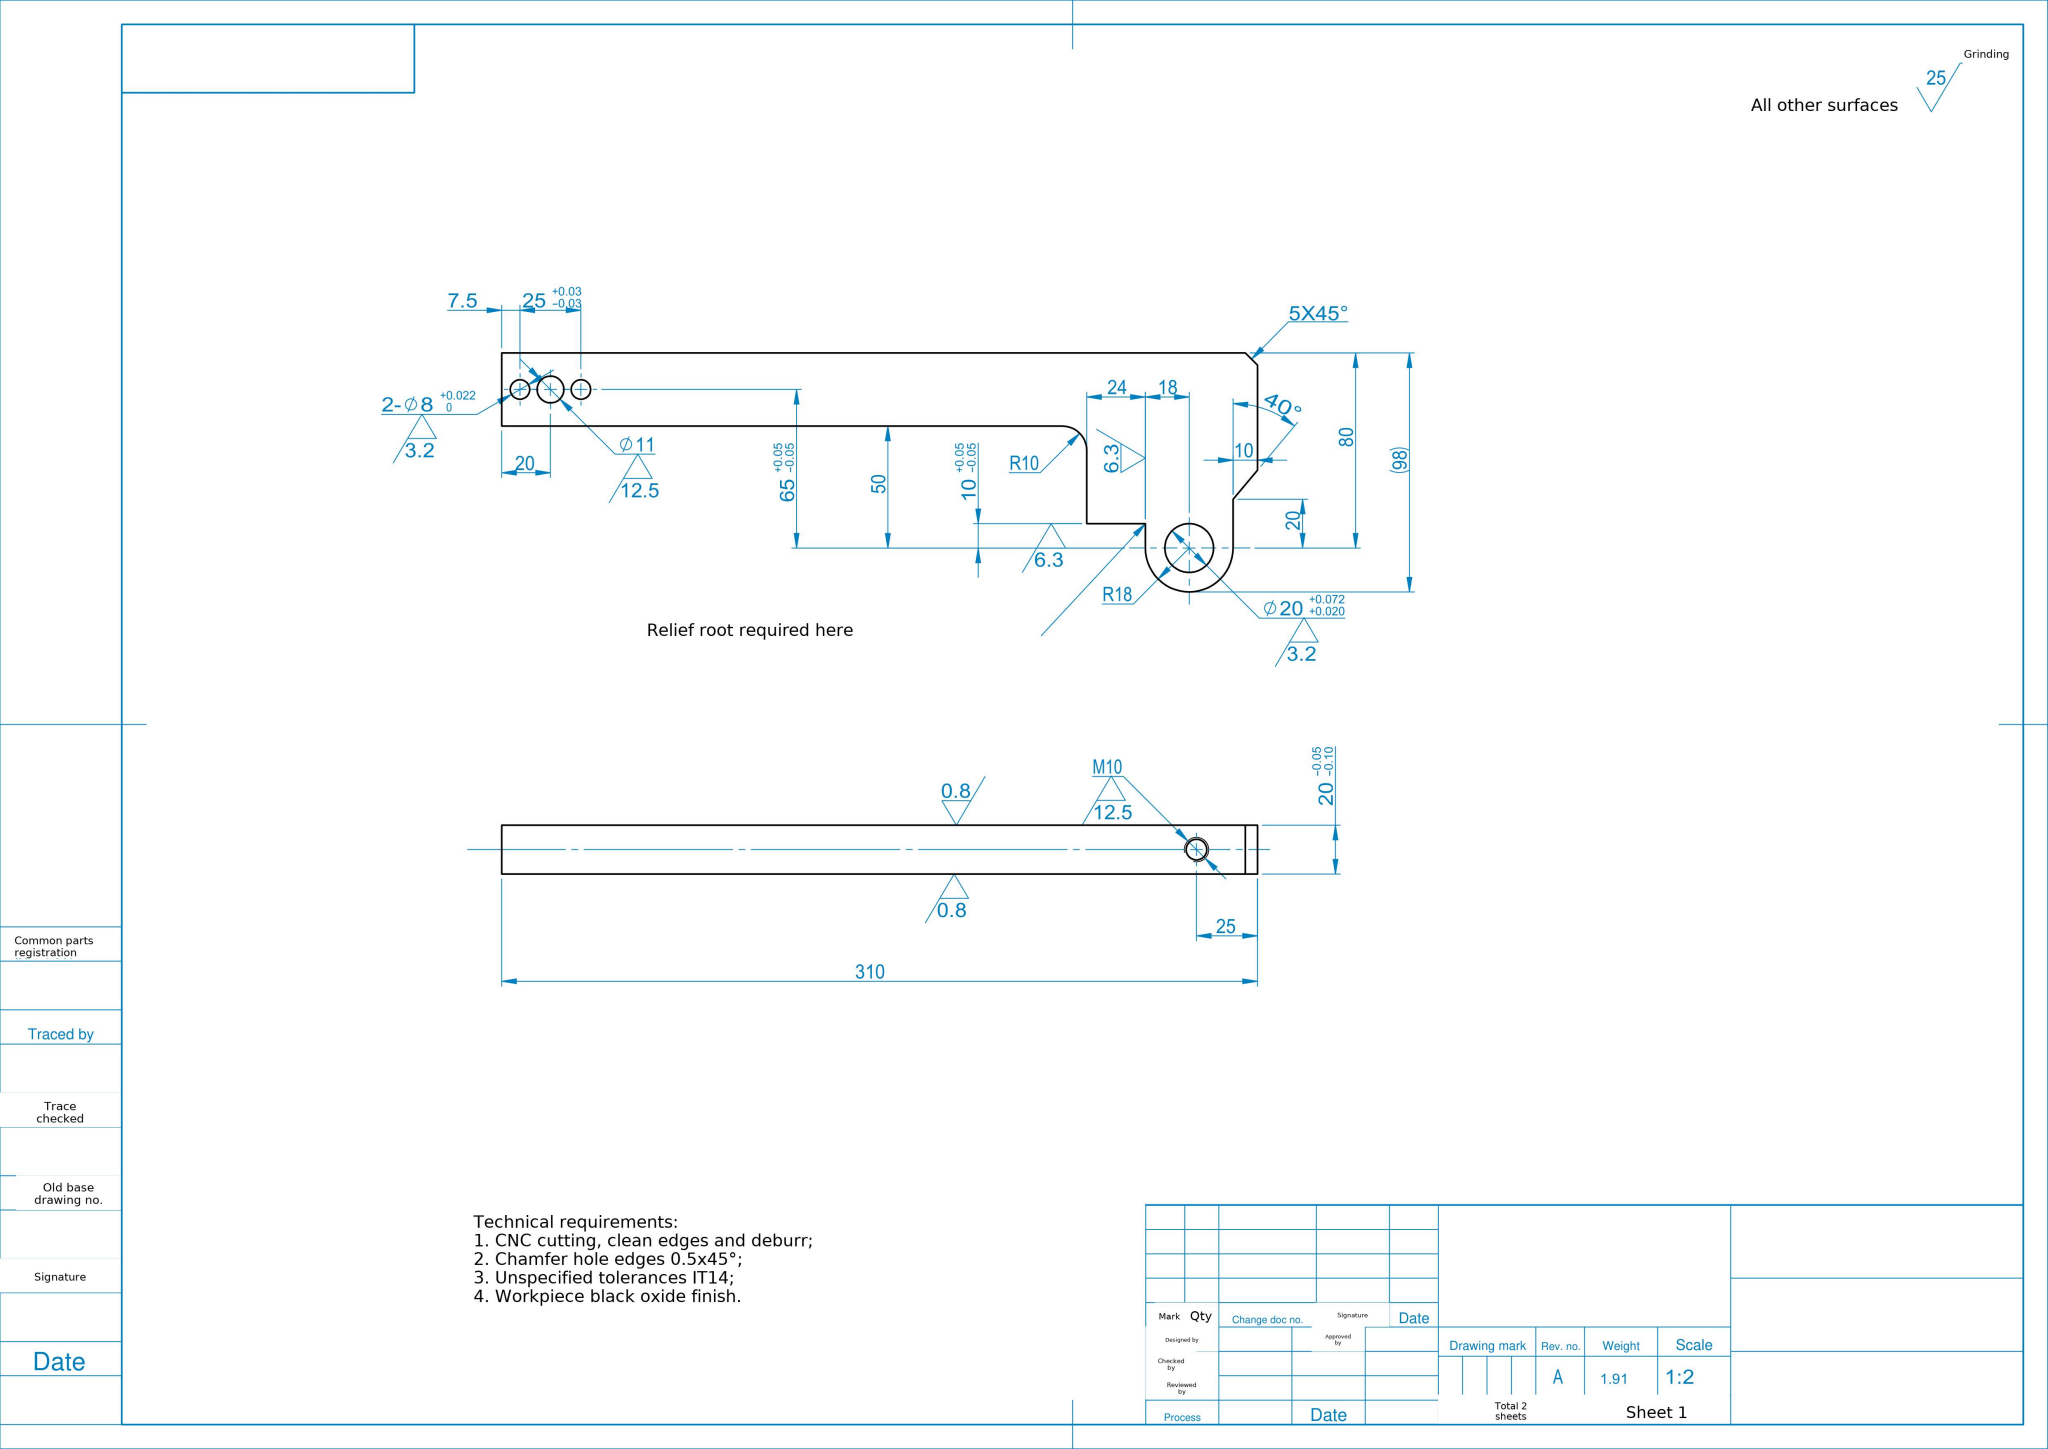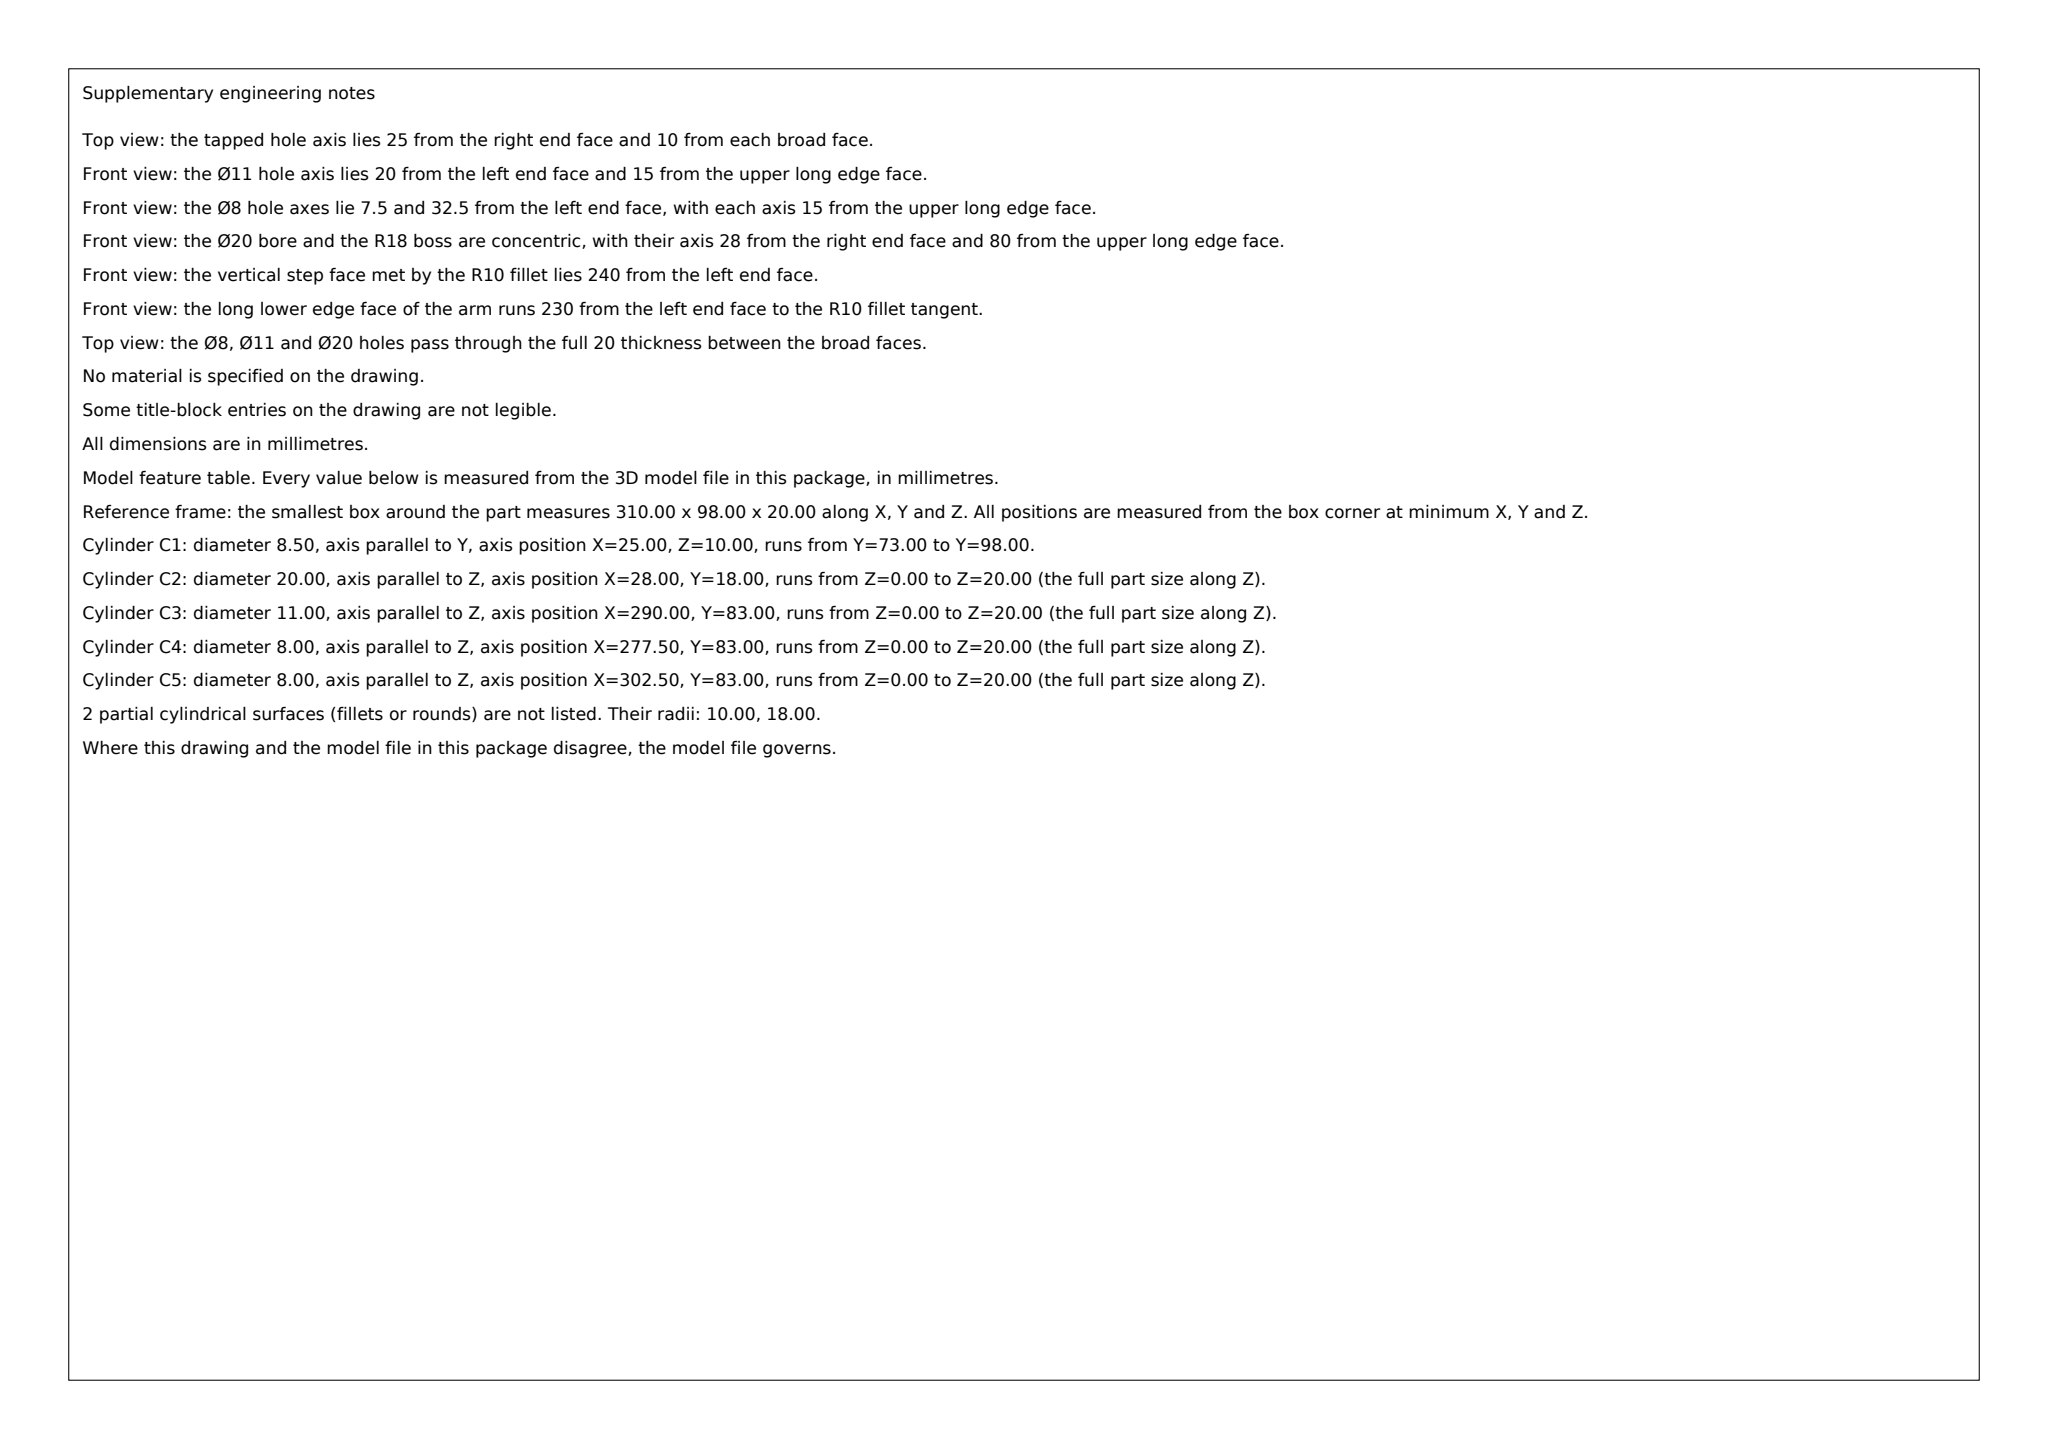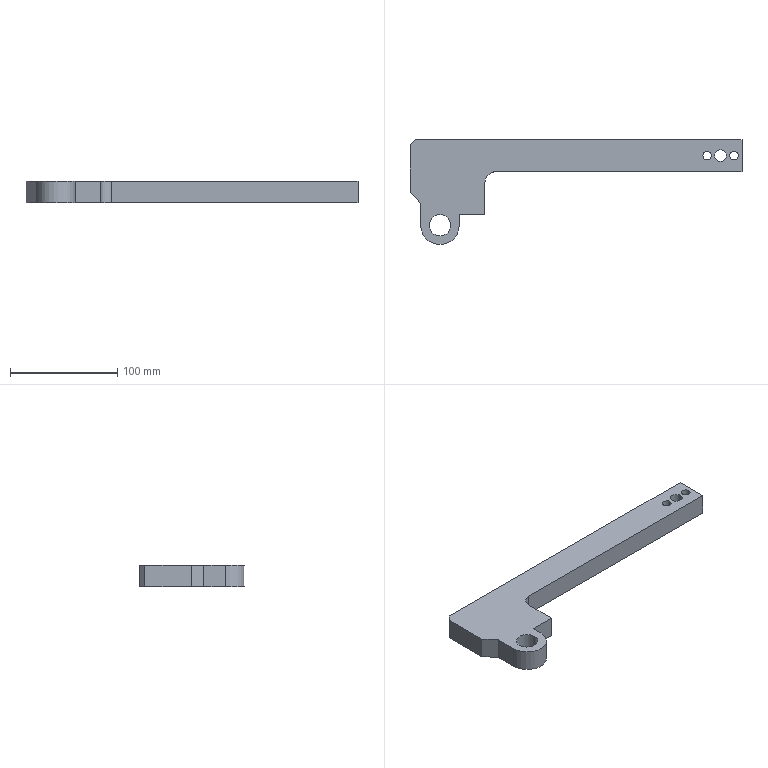Part | SolidWorks | mm | 1 solid | 26 faces | box 310 x 98 x 20 mm | volume 244705 mm3 | cylinder 12 | plane 12 | cone 2 | commonest cylinder face diameters 8 x4 20 x3 11 x2 8.5 x2 36 x1
Drawing notes:
M10 DP 25; Ø8.5 DRILL DP 25, 118° PT (FROM Ø20 BOSS END FACE) | from the solid: cylinder [8.5,"y",[25.0,null,10.0],25.0] blind from y=98 face; cone 118° ref dia 8.5
build123d program:
from build123d import *

# Parameters (mm, degrees)
BOSS_EXTRUDE1_DEPTH    = 20
SKETCH2_R              = 10
CUT_EXTRUDE1_DEPTH     = 319
M10_TAPPED_HOLE1_D     = 8.5
M10_TAPPED_HOLE1_DEPTH = 25
M10_TAPPED_HOLE1_TIP   = 2.554
CHAMFER1_SIZE          = 5
SKETCH8_R              = 5.5
CUT_EXTRUDE2_DEPTH     = 319
SKETCH9_R              = 4
CUT_EXTRUDE3_DEPTH     = 319
FILLET1_R              = 10


with BuildPart() as part:
    # Sketch1 → Boss-Extrude1 (new body)
    with BuildSketch(Plane.XY):
        with BuildLine():
            Line((-264, -40), (-264, -50))
            ThreePointArc((-264, -50), (-282, -68), (-300, -50))
            Line((-300, -50), (-300, -30))
            Line((-300, -30), (-310, -18.082))
            Line((-310, -18.082), (-310, 30))
            Line((-310, 30), (0, 30))
            Line((0, 30), (0, 0))
            Line((0, 0), (-240, 0))
            Line((-240, 0), (-240, -40))
            Line((-240, -40), (-264, -40))
        make_face()
    extrude(amount=BOSS_EXTRUDE1_DEPTH)

    # Sketch2 → Cut-Extrude1 (cut, through all)
    with BuildSketch(Plane(origin=(0, 0, 0), x_dir=(-1, 0, 0), z_dir=(0, 0, -1))):
        with Locations((282, -50)):
            Circle(SKETCH2_R)
    extrude(amount=-CUT_EXTRUDE1_DEPTH, mode=Mode.SUBTRACT)

    # M10 Tapped Hole1
    with Locations(Plane(origin=(0, 30, 0), x_dir=(1, 0, 0), z_dir=(0, 1, 0))):
        with Locations((-285, -10)):
            Hole(M10_TAPPED_HOLE1_D / 2, depth=M10_TAPPED_HOLE1_DEPTH)
            with Locations((0, 0, -(M10_TAPPED_HOLE1_DEPTH + M10_TAPPED_HOLE1_TIP / 2))):  # 118° drill point
                Cone(0, M10_TAPPED_HOLE1_D / 2, M10_TAPPED_HOLE1_TIP, mode=Mode.SUBTRACT)

    # Chamfer1
    chamfer1_edges = [part.edges().sort_by_distance(p)[0] for p in [
        (-310, 30, 10),
    ]]
    chamfer(chamfer1_edges, length=CHAMFER1_SIZE)

    # Sketch8 → Cut-Extrude2 (cut, through all)
    with BuildSketch(Plane(origin=(0, 0, 0), x_dir=(-1, 0, 0), z_dir=(0, 0, -1))):
        with Locations((20, 15)):
            Circle(SKETCH8_R)
    extrude(amount=-CUT_EXTRUDE2_DEPTH, mode=Mode.SUBTRACT)

    # Sketch9 → Cut-Extrude3 (cut, through all)
    with BuildSketch(Plane(origin=(0, 0, 0), x_dir=(-1, 0, 0), z_dir=(0, 0, -1))):
        with Locations((7.5, 15)):
            Circle(SKETCH9_R)
        with Locations((32.5, 15)):
            Circle(SKETCH9_R)
    extrude(amount=-CUT_EXTRUDE3_DEPTH, mode=Mode.SUBTRACT)

    # Fillet1
    fillet1_edges = [part.edges().sort_by_distance(p)[0] for p in [
        (-240, 0, 10),
    ]]
    fillet(fillet1_edges, radius=FILLET1_R)


solid = part.part
STEP:
#1=CARTESIAN_POINT('',(-28.5,15.,20.));
#2=VERTEX_POINT('',#1);
#3=CARTESIAN_POINT('',(-36.5,15.,20.));
#4=VERTEX_POINT('',#3);
#5=CARTESIAN_POINT('',(-32.5,15.,20.));
#6=DIRECTION('',(0.,0.,-1.));
#7=DIRECTION('',(-1.,0.,0.));
#8=AXIS2_PLACEMENT_3D('',#5,#6,#7);
#9=CIRCLE('',#8,4.);
#10=EDGE_CURVE('',#2,#4,#9,.T.);
#11=ORIENTED_EDGE('',*,*,#10,.F.);
#12=CARTESIAN_POINT('',(-28.5,15.,0.));
#13=VERTEX_POINT('',#12);
#14=CARTESIAN_POINT('',(-28.5,15.,20.));
#15=DIRECTION('',(0.,0.,-1.));
#16=VECTOR('',#15,1000.);
#17=LINE('',#14,#16);
#18=EDGE_CURVE('',#2,#13,#17,.T.);
#19=ORIENTED_EDGE('',*,*,#18,.T.);
#20=CARTESIAN_POINT('',(-36.5,15.,0.));
#21=VERTEX_POINT('',#20);
#22=CARTESIAN_POINT('',(-32.5,15.,0.));
#23=DIRECTION('',(0.,0.,-1.));
#24=DIRECTION('',(-1.,0.,0.));
#25=AXIS2_PLACEMENT_3D('',#22,#23,#24);
#26=CIRCLE('',#25,4.);
#27=EDGE_CURVE('',#13,#21,#26,.T.);
#28=ORIENTED_EDGE('',*,*,#27,.T.);
#29=CARTESIAN_POINT('',(-36.5,15.,20.));
#30=DIRECTION('',(0.,0.,-1.));
#31=VECTOR('',#30,1000.);
#32=LINE('',#29,#31);
#33=EDGE_CURVE('',#4,#21,#32,.T.);
#34=ORIENTED_EDGE('',*,*,#33,.F.);
#35=EDGE_LOOP('',(#11,#19,#28,#34));
#36=FACE_OUTER_BOUND('',#35,.T.);
#37=CARTESIAN_POINT('',(-32.5,15.,20.));
#38=DIRECTION('',(0.,0.,-1.));
#39=DIRECTION('',(-1.,0.,0.));
#40=AXIS2_PLACEMENT_3D('',#37,#38,#39);
#41=CYLINDRICAL_SURFACE('',#40,4.);
#42=ADVANCED_FACE('',(#36),#41,.F.);
#43=CARTESIAN_POINT('',(-3.5,15.,20.));
#44=VERTEX_POINT('',#43);
#45=CARTESIAN_POINT('',(-11.5,15.,20.));
#46=VERTEX_POINT('',#45);
#47=CARTESIAN_POINT('',(-7.5,15.,20.));
#48=DIRECTION('',(0.,0.,-1.));
#49=DIRECTION('',(-1.,0.,0.));
#50=AXIS2_PLACEMENT_3D('',#47,#48,#49);
#51=CIRCLE('',#50,4.);
#52=EDGE_CURVE('',#44,#46,#51,.T.);
#53=ORIENTED_EDGE('',*,*,#52,.F.);
#54=CARTESIAN_POINT('',(-3.5,15.,0.));
#55=VERTEX_POINT('',#54);
#56=CARTESIAN_POINT('',(-3.5,15.,20.));
#57=DIRECTION('',(0.,0.,-1.));
#58=VECTOR('',#57,1000.);
#59=LINE('',#56,#58);
#60=EDGE_CURVE('',#44,#55,#59,.T.);
#61=ORIENTED_EDGE('',*,*,#60,.T.);
#62=CARTESIAN_POINT('',(-11.5,15.,0.));
#63=VERTEX_POINT('',#62);
#64=CARTESIAN_POINT('',(-7.5,15.,0.));
#65=DIRECTION('',(0.,0.,-1.));
#66=DIRECTION('',(-1.,0.,0.));
#67=AXIS2_PLACEMENT_3D('',#64,#65,#66);
#68=CIRCLE('',#67,4.);
#69=EDGE_CURVE('',#55,#63,#68,.T.);
#70=ORIENTED_EDGE('',*,*,#69,.T.);
#71=CARTESIAN_POINT('',(-11.5,15.,20.));
#72=DIRECTION('',(0.,0.,-1.));
#73=VECTOR('',#72,1000.);
#74=LINE('',#71,#73);
#75=EDGE_CURVE('',#46,#63,#74,.T.);
#76=ORIENTED_EDGE('',*,*,#75,.F.);
#77=EDGE_LOOP('',(#53,#61,#70,#76));
#78=FACE_OUTER_BOUND('',#77,.T.);
#79=CARTESIAN_POINT('',(-7.5,15.,20.));
#80=DIRECTION('',(0.,0.,-1.));
#81=DIRECTION('',(-1.,0.,0.));
#82=AXIS2_PLACEMENT_3D('',#79,#80,#81);
#83=CYLINDRICAL_SURFACE('',#82,4.);
#84=ADVANCED_FACE('',(#78),#83,.F.);
#85=CARTESIAN_POINT('',(-14.5,15.,20.));
#86=VERTEX_POINT('',#85);
#87=CARTESIAN_POINT('',(-25.5,15.,20.));
#88=VERTEX_POINT('',#87);
#89=CARTESIAN_POINT('',(-20.,15.,20.));
#90=DIRECTION('',(0.,0.,-1.));
#91=DIRECTION('',(-1.,0.,0.));
#92=AXIS2_PLACEMENT_3D('',#89,#90,#91);
#93=CIRCLE('',#92,5.5);
#94=EDGE_CURVE('',#86,#88,#93,.T.);
#95=ORIENTED_EDGE('',*,*,#94,.F.);
#96=CARTESIAN_POINT('',(-14.5,15.,0.));
#97=VERTEX_POINT('',#96);
#98=CARTESIAN_POINT('',(-14.5,15.,20.));
#99=DIRECTION('',(0.,0.,-1.));
#100=VECTOR('',#99,1000.);
#101=LINE('',#98,#100);
#102=EDGE_CURVE('',#86,#97,#101,.T.);
#103=ORIENTED_EDGE('',*,*,#102,.T.);
#104=CARTESIAN_POINT('',(-25.5,15.,0.));
#105=VERTEX_POINT('',#104);
#106=CARTESIAN_POINT('',(-20.,15.,0.));
#107=DIRECTION('',(0.,0.,-1.));
#108=DIRECTION('',(-1.,0.,0.));
#109=AXIS2_PLACEMENT_3D('',#106,#107,#108);
#110=CIRCLE('',#109,5.5);
#111=EDGE_CURVE('',#97,#105,#110,.T.);
#112=ORIENTED_EDGE('',*,*,#111,.T.);
#113=CARTESIAN_POINT('',(-25.5,15.,20.));
#114=DIRECTION('',(0.,0.,-1.));
#115=VECTOR('',#114,1000.);
#116=LINE('',#113,#115);
#117=EDGE_CURVE('',#88,#105,#116,.T.);
#118=ORIENTED_EDGE('',*,*,#117,.F.);
#119=EDGE_LOOP('',(#95,#103,#112,#118));
#120=FACE_OUTER_BOUND('',#119,.T.);
#121=CARTESIAN_POINT('',(-20.,15.,20.));
#122=DIRECTION('',(0.,0.,-1.));
#123=DIRECTION('',(-1.,0.,0.));
#124=AXIS2_PLACEMENT_3D('',#121,#122,#123);
#125=CYLINDRICAL_SURFACE('',#124,5.5);
#126=ADVANCED_FACE('',(#120),#125,.F.);
#127=CARTESIAN_POINT('',(-285.,5.,5.75));
#128=VERTEX_POINT('',#127);
#129=CARTESIAN_POINT('',(-285.,5.,14.25));
#130=VERTEX_POINT('',#129);
#131=CARTESIAN_POINT('',(-285.,5.,10.));
#132=DIRECTION('',(0.,1.,0.));
#133=DIRECTION('',(0.,0.,1.));
#134=AXIS2_PLACEMENT_3D('',#131,#132,#133);
#135=CIRCLE('',#134,4.25);
#136=EDGE_CURVE('',#128,#130,#135,.T.);
#137=ORIENTED_EDGE('',*,*,#136,.F.);
#138=CARTESIAN_POINT('',(-285.,30.,5.75));
#139=VERTEX_POINT('',#138);
#140=CARTESIAN_POINT('',(-285.,30.,5.75));
#141=DIRECTION('',(0.,1.,0.));
#142=VECTOR('',#141,1000.);
#143=LINE('',#140,#142);
#144=EDGE_CURVE('',#128,#139,#143,.T.);
#145=ORIENTED_EDGE('',*,*,#144,.T.);
#146=CARTESIAN_POINT('',(-285.,30.,14.25));
#147=VERTEX_POINT('',#146);
#148=CARTESIAN_POINT('',(-285.,30.,10.));
#149=DIRECTION('',(0.,1.,0.));
#150=DIRECTION('',(0.,0.,1.));
#151=AXIS2_PLACEMENT_3D('',#148,#149,#150);
#152=CIRCLE('',#151,4.25);
#153=EDGE_CURVE('',#139,#147,#152,.T.);
#154=ORIENTED_EDGE('',*,*,#153,.T.);
#155=CARTESIAN_POINT('',(-285.,30.,14.25));
#156=DIRECTION('',(0.,1.,0.));
#157=VECTOR('',#156,1000.);
#158=LINE('',#155,#157);
#159=EDGE_CURVE('',#130,#147,#158,.T.);
#160=ORIENTED_EDGE('',*,*,#159,.F.);
#161=EDGE_LOOP('',(#137,#145,#154,#160));
#162=FACE_OUTER_BOUND('',#161,.T.);
#163=CARTESIAN_POINT('',(-285.,30.,10.));
#164=DIRECTION('',(0.,1.,0.));
#165=DIRECTION('',(0.,0.,1.));
#166=AXIS2_PLACEMENT_3D('',#163,#164,#165);
#167=CYLINDRICAL_SURFACE('',#166,4.25);
#168=ADVANCED_FACE('',(#162),#167,.F.);
#169=CARTESIAN_POINT('',(-285.,2.446,10.));
#170=VERTEX_POINT('',#169);
#171=CARTESIAN_POINT('',(-285.,5.,14.25));
#172=DIRECTION('',(0.,0.515,0.8572));
#173=VECTOR('',#172,1000.);
#174=LINE('',#171,#173);
#175=EDGE_CURVE('',#170,#130,#174,.T.);
#176=ORIENTED_EDGE('',*,*,#175,.F.);
#177=CARTESIAN_POINT('',(-285.,5.,5.75));
#178=DIRECTION('',(0.,0.515,-0.8572));
#179=VECTOR('',#178,1000.);
#180=LINE('',#177,#179);
#181=EDGE_CURVE('',#170,#128,#180,.T.);
#182=ORIENTED_EDGE('',*,*,#181,.T.);
#183=ORIENTED_EDGE('',*,*,#136,.T.);
#184=EDGE_LOOP('',(#176,#182,#183));
#185=FACE_OUTER_BOUND('',#184,.T.);
#186=CARTESIAN_POINT('',(-285.,5.,10.));
#187=DIRECTION('',(0.,1.,0.));
#188=DIRECTION('',(0.,0.,1.));
#189=AXIS2_PLACEMENT_3D('',#186,#187,#188);
#190=CONICAL_SURFACE('',#189,4.25,1.03);
#191=ADVANCED_FACE('',(#185),#190,.F.);
#192=CARTESIAN_POINT('',(-272.,-50.,20.));
#193=VERTEX_POINT('',#192);
#194=CARTESIAN_POINT('',(-292.,-50.,20.));
#195=VERTEX_POINT('',#194);
#196=CARTESIAN_POINT('',(-282.,-50.,20.));
#197=DIRECTION('',(0.,0.,-1.));
#198=DIRECTION('',(-1.,0.,0.));
#199=AXIS2_PLACEMENT_3D('',#196,#197,#198);
#200=CIRCLE('',#199,10.);
#201=EDGE_CURVE('',#193,#195,#200,.T.);
#202=ORIENTED_EDGE('',*,*,#201,.F.);
#203=CARTESIAN_POINT('',(-272.,-50.,0.));
#204=VERTEX_POINT('',#203);
#205=CARTESIAN_POINT('',(-272.,-50.,20.));
#206=DIRECTION('',(0.,0.,-1.));
#207=VECTOR('',#206,1000.);
#208=LINE('',#205,#207);
#209=EDGE_CURVE('',#193,#204,#208,.T.);
#210=ORIENTED_EDGE('',*,*,#209,.T.);
#211=CARTESIAN_POINT('',(-292.,-50.,0.));
#212=VERTEX_POINT('',#211);
#213=CARTESIAN_POINT('',(-282.,-50.,0.));
#214=DIRECTION('',(0.,0.,-1.));
#215=DIRECTION('',(-1.,0.,0.));
#216=AXIS2_PLACEMENT_3D('',#213,#214,#215);
#217=CIRCLE('',#216,10.);
#218=EDGE_CURVE('',#204,#212,#217,.T.);
#219=ORIENTED_EDGE('',*,*,#218,.T.);
#220=CARTESIAN_POINT('',(-292.,-50.,20.));
#221=DIRECTION('',(0.,0.,-1.));
#222=VECTOR('',#221,1000.);
#223=LINE('',#220,#222);
#224=EDGE_CURVE('',#195,#212,#223,.T.);
#225=ORIENTED_EDGE('',*,*,#224,.F.);
#226=EDGE_LOOP('',(#202,#210,#219,#225));
#227=FACE_OUTER_BOUND('',#226,.T.);
#228=CARTESIAN_POINT('',(-282.,-50.,20.));
#229=DIRECTION('',(0.,0.,-1.));
#230=DIRECTION('',(-1.,0.,0.));
#231=AXIS2_PLACEMENT_3D('',#228,#229,#230);
#232=CYLINDRICAL_SURFACE('',#231,10.);
#233=ADVANCED_FACE('',(#227),#232,.F.);
#234=CARTESIAN_POINT('',(0.,0.,0.));
#235=VERTEX_POINT('',#234);
#236=CARTESIAN_POINT('',(0.,30.,0.));
#237=VERTEX_POINT('',#236);
#238=CARTESIAN_POINT('',(0.,0.,0.));
#239=DIRECTION('',(0.,1.,0.));
#240=VECTOR('',#239,1000.);
#241=LINE('',#238,#240);
#242=EDGE_CURVE('',#235,#237,#241,.T.);
#243=ORIENTED_EDGE('',*,*,#242,.T.);
#244=CARTESIAN_POINT('',(0.,30.,20.));
#245=VERTEX_POINT('',#244);
#246=CARTESIAN_POINT('',(0.,30.,20.));
#247=DIRECTION('',(0.,0.,-1.));
#248=VECTOR('',#247,1000.);
#249=LINE('',#246,#248);
#250=EDGE_CURVE('',#245,#237,#249,.T.);
#251=ORIENTED_EDGE('',*,*,#250,.F.);
#252=CARTESIAN_POINT('',(0.,0.,20.));
#253=VERTEX_POINT('',#252);
#254=CARTESIAN_POINT('',(0.,0.,20.));
#255=DIRECTION('',(0.,1.,0.));
#256=VECTOR('',#255,1000.);
#257=LINE('',#254,#256);
#258=EDGE_CURVE('',#253,#245,#257,.T.);
#259=ORIENTED_EDGE('',*,*,#258,.F.);
#260=CARTESIAN_POINT('',(0.,0.,20.));
#261=DIRECTION('',(0.,0.,-1.));
#262=VECTOR('',#261,1000.);
#263=LINE('',#260,#262);
#264=EDGE_CURVE('',#253,#235,#263,.T.);
#265=ORIENTED_EDGE('',*,*,#264,.T.);
#266=EDGE_LOOP('',(#243,#251,#259,#265));
#267=FACE_OUTER_BOUND('',#266,.T.);
#268=CARTESIAN_POINT('',(0.,0.,20.));
#269=DIRECTION('',(-1.,0.,0.));
#270=DIRECTION('',(0.,0.,1.));
#271=AXIS2_PLACEMENT_3D('',#268,#269,#270);
#272=PLANE('',#271);
#273=ADVANCED_FACE('',(#267),#272,.F.);
#274=CARTESIAN_POINT('',(-285.,30.,10.));
#275=DIRECTION('',(0.,1.,0.));
#276=DIRECTION('',(0.,0.,1.));
#277=AXIS2_PLACEMENT_3D('',#274,#275,#276);
#278=CIRCLE('',#277,4.25);
#279=EDGE_CURVE('',#147,#139,#278,.T.);
#280=ORIENTED_EDGE('',*,*,#279,.F.);
#281=ORIENTED_EDGE('',*,*,#153,.F.);
#282=EDGE_LOOP('',(#280,#281));
#283=FACE_BOUND('',#282,.T.);
#284=CARTESIAN_POINT('',(-305.,30.,0.));
#285=VERTEX_POINT('',#284);
#286=CARTESIAN_POINT('',(0.,30.,0.));
#287=DIRECTION('',(-1.,-0.,0.));
#288=VECTOR('',#287,1000.);
#289=LINE('',#286,#288);
#290=EDGE_CURVE('',#237,#285,#289,.T.);
#291=ORIENTED_EDGE('',*,*,#290,.T.);
#292=CARTESIAN_POINT('',(-305.,30.,20.));
#293=VERTEX_POINT('',#292);
#294=CARTESIAN_POINT('',(-305.,30.,20.));
#295=DIRECTION('',(0.,0.,1.));
#296=VECTOR('',#295,1000.);
#297=LINE('',#294,#296);
#298=EDGE_CURVE('',#285,#293,#297,.T.);
#299=ORIENTED_EDGE('',*,*,#298,.T.);
#300=CARTESIAN_POINT('',(0.,30.,20.));
#301=DIRECTION('',(-1.,-0.,0.));
#302=VECTOR('',#301,1000.);
#303=LINE('',#300,#302);
#304=EDGE_CURVE('',#245,#293,#303,.T.);
#305=ORIENTED_EDGE('',*,*,#304,.F.);
#306=ORIENTED_EDGE('',*,*,#250,.T.);
#307=EDGE_LOOP('',(#291,#299,#305,#306));
#308=FACE_OUTER_BOUND('',#307,.T.);
#309=CARTESIAN_POINT('',(0.,30.,20.));
#310=DIRECTION('',(0.,-1.,0.));
#311=DIRECTION('',(1.,0.,0.));
#312=AXIS2_PLACEMENT_3D('',#309,#310,#311);
#313=PLANE('',#312);
#314=ADVANCED_FACE('',(#283,#308),#313,.F.);
#315=CARTESIAN_POINT('',(-310.,25.,20.));
#316=VERTEX_POINT('',#315);
#317=CARTESIAN_POINT('',(-310.,-18.082,20.));
#318=VERTEX_POINT('',#317);
#319=CARTESIAN_POINT('',(-310.,30.,20.));
#320=DIRECTION('',(0.,-1.,0.));
#321=VECTOR('',#320,1000.);
#322=LINE('',#319,#321);
#323=EDGE_CURVE('',#316,#318,#322,.T.);
#324=ORIENTED_EDGE('',*,*,#323,.F.);
#325=CARTESIAN_POINT('',(-310.,25.,0.));
#326=VERTEX_POINT('',#325);
#327=CARTESIAN_POINT('',(-310.,25.,20.));
#328=DIRECTION('',(0.,0.,-1.));
#329=VECTOR('',#328,1000.);
#330=LINE('',#327,#329);
#331=EDGE_CURVE('',#316,#326,#330,.T.);
#332=ORIENTED_EDGE('',*,*,#331,.T.);
#333=CARTESIAN_POINT('',(-310.,-18.082,0.));
#334=VERTEX_POINT('',#333);
#335=CARTESIAN_POINT('',(-310.,30.,0.));
#336=DIRECTION('',(0.,-1.,0.));
#337=VECTOR('',#336,1000.);
#338=LINE('',#335,#337);
#339=EDGE_CURVE('',#326,#334,#338,.T.);
#340=ORIENTED_EDGE('',*,*,#339,.T.);
#341=CARTESIAN_POINT('',(-310.,-18.082,20.));
#342=DIRECTION('',(0.,0.,-1.));
#343=VECTOR('',#342,1000.);
#344=LINE('',#341,#343);
#345=EDGE_CURVE('',#318,#334,#344,.T.);
#346=ORIENTED_EDGE('',*,*,#345,.F.);
#347=EDGE_LOOP('',(#324,#332,#340,#346));
#348=FACE_OUTER_BOUND('',#347,.T.);
#349=CARTESIAN_POINT('',(-310.,30.,20.));
#350=DIRECTION('',(1.,0.,0.));
#351=DIRECTION('',(0.,0.,-1.));
#352=AXIS2_PLACEMENT_3D('',#349,#350,#351);
#353=PLANE('',#352);
#354=ADVANCED_FACE('',(#348),#353,.F.);
#355=CARTESIAN_POINT('',(-300.,-30.,0.));
#356=VERTEX_POINT('',#355);
#357=CARTESIAN_POINT('',(-300.,-30.,0.));
#358=DIRECTION('',(0.6428,-0.766,0.));
#359=VECTOR('',#358,1000.);
#360=LINE('',#357,#359);
#361=EDGE_CURVE('',#334,#356,#360,.T.);
#362=ORIENTED_EDGE('',*,*,#361,.T.);
#363=CARTESIAN_POINT('',(-300.,-30.,20.));
#364=VERTEX_POINT('',#363);
#365=CARTESIAN_POINT('',(-300.,-30.,20.));
#366=DIRECTION('',(0.,0.,-1.));
#367=VECTOR('',#366,1000.);
#368=LINE('',#365,#367);
#369=EDGE_CURVE('',#364,#356,#368,.T.);
#370=ORIENTED_EDGE('',*,*,#369,.F.);
#371=CARTESIAN_POINT('',(-300.,-30.,20.));
#372=DIRECTION('',(0.6428,-0.766,0.));
#373=VECTOR('',#372,1000.);
#374=LINE('',#371,#373);
#375=EDGE_CURVE('',#318,#364,#374,.T.);
#376=ORIENTED_EDGE('',*,*,#375,.F.);
#377=ORIENTED_EDGE('',*,*,#345,.T.);
#378=EDGE_LOOP('',(#362,#370,#376,#377));
#379=FACE_OUTER_BOUND('',#378,.T.);
#380=CARTESIAN_POINT('',(-300.,-30.,20.));
#381=DIRECTION('',(0.766,0.6428,0.));
#382=DIRECTION('',(-0.6428,0.766,0.));
#383=AXIS2_PLACEMENT_3D('',#380,#381,#382);
#384=PLANE('',#383);
#385=ADVANCED_FACE('',(#379),#384,.F.);
#386=CARTESIAN_POINT('',(-300.,-50.,0.));
#387=VERTEX_POINT('',#386);
#388=CARTESIAN_POINT('',(-300.,-50.,0.));
#389=DIRECTION('',(0.,-1.,0.));
#390=VECTOR('',#389,1000.);
#391=LINE('',#388,#390);
#392=EDGE_CURVE('',#356,#387,#391,.T.);
#393=ORIENTED_EDGE('',*,*,#392,.T.);
#394=CARTESIAN_POINT('',(-300.,-50.,20.));
#395=VERTEX_POINT('',#394);
#396=CARTESIAN_POINT('',(-300.,-50.,20.));
#397=DIRECTION('',(0.,0.,-1.));
#398=VECTOR('',#397,1000.);
#399=LINE('',#396,#398);
#400=EDGE_CURVE('',#395,#387,#399,.T.);
#401=ORIENTED_EDGE('',*,*,#400,.F.);
#402=CARTESIAN_POINT('',(-300.,-50.,20.));
#403=DIRECTION('',(0.,-1.,0.));
#404=VECTOR('',#403,1000.);
#405=LINE('',#402,#404);
#406=EDGE_CURVE('',#364,#395,#405,.T.);
#407=ORIENTED_EDGE('',*,*,#406,.F.);
#408=ORIENTED_EDGE('',*,*,#369,.T.);
#409=EDGE_LOOP('',(#393,#401,#407,#408));
#410=FACE_OUTER_BOUND('',#409,.T.);
#411=CARTESIAN_POINT('',(-300.,-50.,20.));
#412=DIRECTION('',(1.,0.,0.));
#413=DIRECTION('',(0.,0.,-1.));
#414=AXIS2_PLACEMENT_3D('',#411,#412,#413);
#415=PLANE('',#414);
#416=ADVANCED_FACE('',(#410),#415,.F.);
#417=CARTESIAN_POINT('',(-264.,-50.,0.));
#418=VERTEX_POINT('',#417);
#419=CARTESIAN_POINT('',(-282.,-50.,0.));
#420=DIRECTION('',(0.,0.,1.));
#421=DIRECTION('',(1.,0.,0.));
#422=AXIS2_PLACEMENT_3D('',#419,#420,#421);
#423=CIRCLE('',#422,18.);
#424=EDGE_CURVE('',#387,#418,#423,.T.);
#425=ORIENTED_EDGE('',*,*,#424,.T.);
#426=CARTESIAN_POINT('',(-264.,-50.,20.));
#427=VERTEX_POINT('',#426);
#428=CARTESIAN_POINT('',(-264.,-50.,20.));
#429=DIRECTION('',(0.,0.,-1.));
#430=VECTOR('',#429,1000.);
#431=LINE('',#428,#430);
#432=EDGE_CURVE('',#427,#418,#431,.T.);
#433=ORIENTED_EDGE('',*,*,#432,.F.);
#434=CARTESIAN_POINT('',(-282.,-50.,20.));
#435=DIRECTION('',(0.,0.,1.));
#436=DIRECTION('',(1.,0.,0.));
#437=AXIS2_PLACEMENT_3D('',#434,#435,#436);
#438=CIRCLE('',#437,18.);
#439=EDGE_CURVE('',#395,#427,#438,.T.);
#440=ORIENTED_EDGE('',*,*,#439,.F.);
#441=ORIENTED_EDGE('',*,*,#400,.T.);
#442=EDGE_LOOP('',(#425,#433,#440,#441));
#443=FACE_OUTER_BOUND('',#442,.T.);
#444=CARTESIAN_POINT('',(-282.,-50.,20.));
#445=DIRECTION('',(0.,0.,-1.));
#446=DIRECTION('',(-1.,0.,0.));
#447=AXIS2_PLACEMENT_3D('',#444,#445,#446);
#448=CYLINDRICAL_SURFACE('',#447,18.);
#449=ADVANCED_FACE('',(#443),#448,.T.);
#450=CARTESIAN_POINT('',(-264.,-40.,0.));
#451=VERTEX_POINT('',#450);
#452=CARTESIAN_POINT('',(-264.,-40.,0.));
#453=DIRECTION('',(0.,1.,0.));
#454=VECTOR('',#453,1000.);
#455=LINE('',#452,#454);
#456=EDGE_CURVE('',#418,#451,#455,.T.);
#457=ORIENTED_EDGE('',*,*,#456,.T.);
#458=CARTESIAN_POINT('',(-264.,-40.,20.));
#459=VERTEX_POINT('',#458);
#460=CARTESIAN_POINT('',(-264.,-40.,20.));
#461=DIRECTION('',(0.,0.,-1.));
#462=VECTOR('',#461,1000.);
#463=LINE('',#460,#462);
#464=EDGE_CURVE('',#459,#451,#463,.T.);
#465=ORIENTED_EDGE('',*,*,#464,.F.);
#466=CARTESIAN_POINT('',(-264.,-40.,20.));
#467=DIRECTION('',(0.,1.,0.));
#468=VECTOR('',#467,1000.);
#469=LINE('',#466,#468);
#470=EDGE_CURVE('',#427,#459,#469,.T.);
#471=ORIENTED_EDGE('',*,*,#470,.F.);
#472=ORIENTED_EDGE('',*,*,#432,.T.);
#473=EDGE_LOOP('',(#457,#465,#471,#472));
#474=FACE_OUTER_BOUND('',#473,.T.);
#475=CARTESIAN_POINT('',(-264.,-40.,20.));
#476=DIRECTION('',(-1.,0.,0.));
#477=DIRECTION('',(0.,0.,1.));
#478=AXIS2_PLACEMENT_3D('',#475,#476,#477);
#479=PLANE('',#478);
#480=ADVANCED_FACE('',(#474),#479,.F.);
#481=CARTESIAN_POINT('',(-240.,-40.,0.));
#482=VERTEX_POINT('',#481);
#483=CARTESIAN_POINT('',(-240.,-40.,0.));
#484=DIRECTION('',(1.,0.,0.));
#485=VECTOR('',#484,1000.);
#486=LINE('',#483,#485);
#487=EDGE_CURVE('',#451,#482,#486,.T.);
#488=ORIENTED_EDGE('',*,*,#487,.T.);
#489=CARTESIAN_POINT('',(-240.,-40.,20.));
#490=VERTEX_POINT('',#489);
#491=CARTESIAN_POINT('',(-240.,-40.,20.));
#492=DIRECTION('',(0.,0.,-1.));
#493=VECTOR('',#492,1000.);
#494=LINE('',#491,#493);
#495=EDGE_CURVE('',#490,#482,#494,.T.);
#496=ORIENTED_EDGE('',*,*,#495,.F.);
#497=CARTESIAN_POINT('',(-240.,-40.,20.));
#498=DIRECTION('',(1.,0.,0.));
#499=VECTOR('',#498,1000.);
#500=LINE('',#497,#499);
#501=EDGE_CURVE('',#459,#490,#500,.T.);
#502=ORIENTED_EDGE('',*,*,#501,.F.);
#503=ORIENTED_EDGE('',*,*,#464,.T.);
#504=EDGE_LOOP('',(#488,#496,#502,#503));
#505=FACE_OUTER_BOUND('',#504,.T.);
#506=CARTESIAN_POINT('',(-240.,-40.,20.));
#507=DIRECTION('',(-0.,1.,0.));
#508=DIRECTION('',(-1.,-0.,0.));
#509=AXIS2_PLACEMENT_3D('',#506,#507,#508);
#510=PLANE('',#509);
#511=ADVANCED_FACE('',(#505),#510,.F.);
#512=CARTESIAN_POINT('',(-240.,-10.,0.));
#513=VERTEX_POINT('',#512);
#514=CARTESIAN_POINT('',(-240.,-0.,0.));
#515=DIRECTION('',(0.,1.,0.));
#516=VECTOR('',#515,1000.);
#517=LINE('',#514,#516);
#518=EDGE_CURVE('',#482,#513,#517,.T.);
#519=ORIENTED_EDGE('',*,*,#518,.T.);
#520=CARTESIAN_POINT('',(-240.,-10.,20.));
#521=VERTEX_POINT('',#520);
#522=CARTESIAN_POINT('',(-240.,-10.,20.));
#523=DIRECTION('',(0.,0.,1.));
#524=VECTOR('',#523,1000.);
#525=LINE('',#522,#524);
#526=EDGE_CURVE('',#513,#521,#525,.T.);
#527=ORIENTED_EDGE('',*,*,#526,.T.);
#528=CARTESIAN_POINT('',(-240.,-0.,20.));
#529=DIRECTION('',(0.,1.,0.));
#530=VECTOR('',#529,1000.);
#531=LINE('',#528,#530);
#532=EDGE_CURVE('',#490,#521,#531,.T.);
#533=ORIENTED_EDGE('',*,*,#532,.F.);
#534=ORIENTED_EDGE('',*,*,#495,.T.);
#535=EDGE_LOOP('',(#519,#527,#533,#534));
#536=FACE_OUTER_BOUND('',#535,.T.);
#537=CARTESIAN_POINT('',(-240.,-0.,20.));
#538=DIRECTION('',(-1.,0.,0.));
#539=DIRECTION('',(0.,0.,1.));
#540=AXIS2_PLACEMENT_3D('',#537,#538,#539);
#541=PLANE('',#540);
#542=ADVANCED_FACE('',(#536),#541,.F.);
#543=CARTESIAN_POINT('',(-230.,-0.,20.));
#544=VERTEX_POINT('',#543);
#545=CARTESIAN_POINT('',(0.,0.,20.));
#546=DIRECTION('',(1.,0.,0.));
#547=VECTOR('',#546,1000.);
#548=LINE('',#545,#547);
#549=EDGE_CURVE('',#544,#253,#548,.T.);
#550=ORIENTED_EDGE('',*,*,#549,.F.);
#551=CARTESIAN_POINT('',(-230.,-0.,0.));
#552=VERTEX_POINT('',#551);
#553=CARTESIAN_POINT('',(-230.,-0.,0.));
#554=DIRECTION('',(0.,0.,-1.));
#555=VECTOR('',#554,1000.);
#556=LINE('',#553,#555);
#557=EDGE_CURVE('',#544,#552,#556,.T.);
#558=ORIENTED_EDGE('',*,*,#557,.T.);
#559=CARTESIAN_POINT('',(0.,0.,0.));
#560=DIRECTION('',(1.,0.,0.));
#561=VECTOR('',#560,1000.);
#562=LINE('',#559,#561);
#563=EDGE_CURVE('',#552,#235,#562,.T.);
#564=ORIENTED_EDGE('',*,*,#563,.T.);
#565=ORIENTED_EDGE('',*,*,#264,.F.);
#566=EDGE_LOOP('',(#550,#558,#564,#565));
#567=FACE_OUTER_BOUND('',#566,.T.);
#568=CARTESIAN_POINT('',(0.,0.,20.));
#569=DIRECTION('',(-0.,1.,0.));
#570=DIRECTION('',(-1.,-0.,0.));
#571=AXIS2_PLACEMENT_3D('',#568,#569,#570);
#572=PLANE('',#571);
#573=ADVANCED_FACE('',(#567),#572,.F.);
#574=CARTESIAN_POINT('',(-32.5,15.,20.));
#575=DIRECTION('',(0.,0.,-1.));
#576=DIRECTION('',(-1.,0.,0.));
#577=AXIS2_PLACEMENT_3D('',#574,#575,#576);
#578=CIRCLE('',#577,4.);
#579=EDGE_CURVE('',#4,#2,#578,.T.);
#580=ORIENTED_EDGE('',*,*,#579,.T.);
#581=ORIENTED_EDGE('',*,*,#10,.T.);
#582=EDGE_LOOP('',(#580,#581));
#583=FACE_BOUND('',#582,.T.);
#584=CARTESIAN_POINT('',(-7.5,15.,20.));
#585=DIRECTION('',(0.,0.,-1.));
#586=DIRECTION('',(-1.,0.,0.));
#587=AXIS2_PLACEMENT_3D('',#584,#585,#586);
#588=CIRCLE('',#587,4.);
#589=EDGE_CURVE('',#46,#44,#588,.T.);
#590=ORIENTED_EDGE('',*,*,#589,.T.);
#591=ORIENTED_EDGE('',*,*,#52,.T.);
#592=EDGE_LOOP('',(#590,#591));
#593=FACE_BOUND('',#592,.T.);
#594=CARTESIAN_POINT('',(-20.,15.,20.));
#595=DIRECTION('',(0.,0.,-1.));
#596=DIRECTION('',(-1.,0.,0.));
#597=AXIS2_PLACEMENT_3D('',#594,#595,#596);
#598=CIRCLE('',#597,5.5);
#599=EDGE_CURVE('',#88,#86,#598,.T.);
#600=ORIENTED_EDGE('',*,*,#599,.T.);
#601=ORIENTED_EDGE('',*,*,#94,.T.);
#602=EDGE_LOOP('',(#600,#601));
#603=FACE_BOUND('',#602,.T.);
#604=CARTESIAN_POINT('',(-282.,-50.,20.));
#605=DIRECTION('',(0.,0.,-1.));
#606=DIRECTION('',(-1.,0.,0.));
#607=AXIS2_PLACEMENT_3D('',#604,#605,#606);
#608=CIRCLE('',#607,10.);
#609=EDGE_CURVE('',#195,#193,#608,.T.);
#610=ORIENTED_EDGE('',*,*,#609,.T.);
#611=ORIENTED_EDGE('',*,*,#201,.T.);
#612=EDGE_LOOP('',(#610,#611));
#613=FACE_BOUND('',#612,.T.);
#614=ORIENTED_EDGE('',*,*,#304,.T.);
#615=CARTESIAN_POINT('',(-333.5,1.5,20.));
#616=DIRECTION('',(-0.7071,-0.7071,0.));
#617=VECTOR('',#616,1000.);
#618=LINE('',#615,#617);
#619=EDGE_CURVE('',#293,#316,#618,.T.);
#620=ORIENTED_EDGE('',*,*,#619,.T.);
#621=ORIENTED_EDGE('',*,*,#323,.T.);
#622=ORIENTED_EDGE('',*,*,#375,.T.);
#623=ORIENTED_EDGE('',*,*,#406,.T.);
#624=ORIENTED_EDGE('',*,*,#439,.T.);
#625=ORIENTED_EDGE('',*,*,#470,.T.);
#626=ORIENTED_EDGE('',*,*,#501,.T.);
#627=ORIENTED_EDGE('',*,*,#532,.T.);
#628=CARTESIAN_POINT('',(-230.,-10.,20.));
#629=DIRECTION('',(0.,0.,-1.));
#630=DIRECTION('',(1.,0.,0.));
#631=AXIS2_PLACEMENT_3D('',#628,#629,#630);
#632=CIRCLE('',#631,10.);
#633=EDGE_CURVE('',#521,#544,#632,.T.);
#634=ORIENTED_EDGE('',*,*,#633,.T.);
#635=ORIENTED_EDGE('',*,*,#549,.T.);
#636=ORIENTED_EDGE('',*,*,#258,.T.);
#637=EDGE_LOOP('',(#614,#620,#621,#622,#623,#624,#625,#626,#627,#634,#635,#636));
#638=FACE_OUTER_BOUND('',#637,.T.);
#639=CARTESIAN_POINT('',(-282.,-50.,20.));
#640=DIRECTION('',(0.,0.,1.));
#641=DIRECTION('',(1.,0.,0.));
#642=AXIS2_PLACEMENT_3D('',#639,#640,#641);
#643=PLANE('',#642);
#644=ADVANCED_FACE('',(#583,#593,#603,#613,#638),#643,.T.);
#645=CARTESIAN_POINT('',(-32.5,15.,0.));
#646=DIRECTION('',(0.,0.,-1.));
#647=DIRECTION('',(-1.,0.,0.));
#648=AXIS2_PLACEMENT_3D('',#645,#646,#647);
#649=CIRCLE('',#648,4.);
#650=EDGE_CURVE('',#21,#13,#649,.T.);
#651=ORIENTED_EDGE('',*,*,#650,.F.);
#652=ORIENTED_EDGE('',*,*,#27,.F.);
#653=EDGE_LOOP('',(#651,#652));
#654=FACE_BOUND('',#653,.T.);
#655=CARTESIAN_POINT('',(-7.5,15.,0.));
#656=DIRECTION('',(0.,0.,-1.));
#657=DIRECTION('',(-1.,0.,0.));
#658=AXIS2_PLACEMENT_3D('',#655,#656,#657);
#659=CIRCLE('',#658,4.);
#660=EDGE_CURVE('',#63,#55,#659,.T.);
#661=ORIENTED_EDGE('',*,*,#660,.F.);
#662=ORIENTED_EDGE('',*,*,#69,.F.);
#663=EDGE_LOOP('',(#661,#662));
#664=FACE_BOUND('',#663,.T.);
#665=CARTESIAN_POINT('',(-20.,15.,0.));
#666=DIRECTION('',(0.,0.,-1.));
#667=DIRECTION('',(-1.,0.,0.));
#668=AXIS2_PLACEMENT_3D('',#665,#666,#667);
#669=CIRCLE('',#668,5.5);
#670=EDGE_CURVE('',#105,#97,#669,.T.);
#671=ORIENTED_EDGE('',*,*,#670,.F.);
#672=ORIENTED_EDGE('',*,*,#111,.F.);
#673=EDGE_LOOP('',(#671,#672));
#674=FACE_BOUND('',#673,.T.);
#675=CARTESIAN_POINT('',(-282.,-50.,0.));
#676=DIRECTION('',(0.,0.,-1.));
#677=DIRECTION('',(-1.,0.,0.));
#678=AXIS2_PLACEMENT_3D('',#675,#676,#677);
#679=CIRCLE('',#678,10.);
#680=EDGE_CURVE('',#212,#204,#679,.T.);
#681=ORIENTED_EDGE('',*,*,#680,.F.);
#682=ORIENTED_EDGE('',*,*,#218,.F.);
#683=EDGE_LOOP('',(#681,#682));
#684=FACE_BOUND('',#683,.T.);
#685=ORIENTED_EDGE('',*,*,#339,.F.);
#686=CARTESIAN_POINT('',(-310.,25.,0.));
#687=DIRECTION('',(0.7071,0.7071,0.));
#688=VECTOR('',#687,1000.);
#689=LINE('',#686,#688);
#690=EDGE_CURVE('',#326,#285,#689,.T.);
#691=ORIENTED_EDGE('',*,*,#690,.T.);
#692=ORIENTED_EDGE('',*,*,#290,.F.);
#693=ORIENTED_EDGE('',*,*,#242,.F.);
#694=ORIENTED_EDGE('',*,*,#563,.F.);
#695=CARTESIAN_POINT('',(-230.,-10.,0.));
#696=DIRECTION('',(0.,0.,1.));
#697=DIRECTION('',(1.,0.,0.));
#698=AXIS2_PLACEMENT_3D('',#695,#696,#697);
#699=CIRCLE('',#698,10.);
#700=EDGE_CURVE('',#552,#513,#699,.T.);
#701=ORIENTED_EDGE('',*,*,#700,.T.);
#702=ORIENTED_EDGE('',*,*,#518,.F.);
#703=ORIENTED_EDGE('',*,*,#487,.F.);
#704=ORIENTED_EDGE('',*,*,#456,.F.);
#705=ORIENTED_EDGE('',*,*,#424,.F.);
#706=ORIENTED_EDGE('',*,*,#392,.F.);
#707=ORIENTED_EDGE('',*,*,#361,.F.);
#708=EDGE_LOOP('',(#685,#691,#692,#693,#694,#701,#702,#703,#704,#705,#706,#707));
#709=FACE_OUTER_BOUND('',#708,.T.);
#710=CARTESIAN_POINT('',(-282.,-50.,0.));
#711=DIRECTION('',(0.,0.,1.));
#712=DIRECTION('',(1.,0.,0.));
#713=AXIS2_PLACEMENT_3D('',#710,#711,#712);
#714=PLANE('',#713);
#715=ADVANCED_FACE('',(#654,#664,#674,#684,#709),#714,.F.);
#716=ORIENTED_EDGE('',*,*,#209,.F.);
#717=ORIENTED_EDGE('',*,*,#609,.F.);
#718=ORIENTED_EDGE('',*,*,#224,.T.);
#719=ORIENTED_EDGE('',*,*,#680,.T.);
#720=EDGE_LOOP('',(#716,#717,#718,#719));
#721=FACE_OUTER_BOUND('',#720,.T.);
#722=CARTESIAN_POINT('',(-282.,-50.,20.));
#723=DIRECTION('',(0.,0.,-1.));
#724=DIRECTION('',(-1.,0.,0.));
#725=AXIS2_PLACEMENT_3D('',#722,#723,#724);
#726=CYLINDRICAL_SURFACE('',#725,10.);
#727=ADVANCED_FACE('',(#721),#726,.F.);
#728=ORIENTED_EDGE('',*,*,#181,.F.);
#729=ORIENTED_EDGE('',*,*,#175,.T.);
#730=CARTESIAN_POINT('',(-285.,5.,10.));
#731=DIRECTION('',(0.,1.,0.));
#732=DIRECTION('',(0.,0.,1.));
#733=AXIS2_PLACEMENT_3D('',#730,#731,#732);
#734=CIRCLE('',#733,4.25);
#735=EDGE_CURVE('',#130,#128,#734,.T.);
#736=ORIENTED_EDGE('',*,*,#735,.T.);
#737=EDGE_LOOP('',(#728,#729,#736));
#738=FACE_OUTER_BOUND('',#737,.T.);
#739=CARTESIAN_POINT('',(-285.,5.,10.));
#740=DIRECTION('',(0.,1.,0.));
#741=DIRECTION('',(0.,0.,1.));
#742=AXIS2_PLACEMENT_3D('',#739,#740,#741);
#743=CONICAL_SURFACE('',#742,4.25,1.03);
#744=ADVANCED_FACE('',(#738),#743,.F.);
#745=ORIENTED_EDGE('',*,*,#144,.F.);
#746=ORIENTED_EDGE('',*,*,#735,.F.);
#747=ORIENTED_EDGE('',*,*,#159,.T.);
#748=ORIENTED_EDGE('',*,*,#279,.T.);
#749=EDGE_LOOP('',(#745,#746,#747,#748));
#750=FACE_OUTER_BOUND('',#749,.T.);
#751=CARTESIAN_POINT('',(-285.,30.,10.));
#752=DIRECTION('',(0.,1.,0.));
#753=DIRECTION('',(0.,0.,1.));
#754=AXIS2_PLACEMENT_3D('',#751,#752,#753);
#755=CYLINDRICAL_SURFACE('',#754,4.25);
#756=ADVANCED_FACE('',(#750),#755,.F.);
#757=ORIENTED_EDGE('',*,*,#619,.F.);
#758=ORIENTED_EDGE('',*,*,#298,.F.);
#759=ORIENTED_EDGE('',*,*,#690,.F.);
#760=ORIENTED_EDGE('',*,*,#331,.F.);
#761=EDGE_LOOP('',(#757,#758,#759,#760));
#762=FACE_OUTER_BOUND('',#761,.T.);
#763=CARTESIAN_POINT('',(-310.,25.,20.));
#764=DIRECTION('',(0.7071,-0.7071,0.));
#765=DIRECTION('',(0.,0.,-1.));
#766=AXIS2_PLACEMENT_3D('',#763,#764,#765);
#767=PLANE('',#766);
#768=ADVANCED_FACE('',(#762),#767,.F.);
#769=ORIENTED_EDGE('',*,*,#102,.F.);
#770=ORIENTED_EDGE('',*,*,#599,.F.);
#771=ORIENTED_EDGE('',*,*,#117,.T.);
#772=ORIENTED_EDGE('',*,*,#670,.T.);
#773=EDGE_LOOP('',(#769,#770,#771,#772));
#774=FACE_OUTER_BOUND('',#773,.T.);
#775=CARTESIAN_POINT('',(-20.,15.,20.));
#776=DIRECTION('',(0.,0.,-1.));
#777=DIRECTION('',(-1.,0.,0.));
#778=AXIS2_PLACEMENT_3D('',#775,#776,#777);
#779=CYLINDRICAL_SURFACE('',#778,5.5);
#780=ADVANCED_FACE('',(#774),#779,.F.);
#781=ORIENTED_EDGE('',*,*,#60,.F.);
#782=ORIENTED_EDGE('',*,*,#589,.F.);
#783=ORIENTED_EDGE('',*,*,#75,.T.);
#784=ORIENTED_EDGE('',*,*,#660,.T.);
#785=EDGE_LOOP('',(#781,#782,#783,#784));
#786=FACE_OUTER_BOUND('',#785,.T.);
#787=CARTESIAN_POINT('',(-7.5,15.,20.));
#788=DIRECTION('',(0.,0.,-1.));
#789=DIRECTION('',(-1.,0.,0.));
#790=AXIS2_PLACEMENT_3D('',#787,#788,#789);
#791=CYLINDRICAL_SURFACE('',#790,4.);
#792=ADVANCED_FACE('',(#786),#791,.F.);
#793=ORIENTED_EDGE('',*,*,#18,.F.);
#794=ORIENTED_EDGE('',*,*,#579,.F.);
#795=ORIENTED_EDGE('',*,*,#33,.T.);
#796=ORIENTED_EDGE('',*,*,#650,.T.);
#797=EDGE_LOOP('',(#793,#794,#795,#796));
#798=FACE_OUTER_BOUND('',#797,.T.);
#799=CARTESIAN_POINT('',(-32.5,15.,20.));
#800=DIRECTION('',(0.,0.,-1.));
#801=DIRECTION('',(-1.,0.,0.));
#802=AXIS2_PLACEMENT_3D('',#799,#800,#801);
#803=CYLINDRICAL_SURFACE('',#802,4.);
#804=ADVANCED_FACE('',(#798),#803,.F.);
#805=ORIENTED_EDGE('',*,*,#633,.F.);
#806=ORIENTED_EDGE('',*,*,#526,.F.);
#807=ORIENTED_EDGE('',*,*,#700,.F.);
#808=ORIENTED_EDGE('',*,*,#557,.F.);
#809=EDGE_LOOP('',(#805,#806,#807,#808));
#810=FACE_OUTER_BOUND('',#809,.T.);
#811=CARTESIAN_POINT('',(-230.,-10.,20.));
#812=DIRECTION('',(0.,0.,1.));
#813=DIRECTION('',(1.,0.,0.));
#814=AXIS2_PLACEMENT_3D('',#811,#812,#813);
#815=CYLINDRICAL_SURFACE('',#814,10.);
#816=ADVANCED_FACE('',(#810),#815,.F.);
#817=CLOSED_SHELL('',(#42,#84,#126,#168,#191,#233,#273,#314,#354,#385,#416,#449,#480,#511,#542,#573,#644,#715,#727,#744,#756,#768,#780,#792,#804,#816));
#818=MANIFOLD_SOLID_BREP('',#817);
#819=CARTESIAN_POINT('',(0.,0.,0.));
#820=DIRECTION('',(0.,0.,1.));
#821=DIRECTION('',(1.,0.,0.));
#822=AXIS2_PLACEMENT_3D('',#819,#820,#821);
#823=(LENGTH_UNIT()NAMED_UNIT(*)SI_UNIT(.MILLI.,.METRE.));
#824=UNCERTAINTY_MEASURE_WITH_UNIT(LENGTH_MEASURE(0.00001),#823,'','');
#825=(NAMED_UNIT(*)PLANE_ANGLE_UNIT()SI_UNIT($,.RADIAN.));
#826=(NAMED_UNIT(*)SI_UNIT($,.STERADIAN.)SOLID_ANGLE_UNIT());
#827=(GEOMETRIC_REPRESENTATION_CONTEXT(3)GLOBAL_UNCERTAINTY_ASSIGNED_CONTEXT((#824))GLOBAL_UNIT_ASSIGNED_CONTEXT((#823,#825,#826))REPRESENTATION_CONTEXT('',''));
#828=ADVANCED_BREP_SHAPE_REPRESENTATION('',(#818,#822),#827);